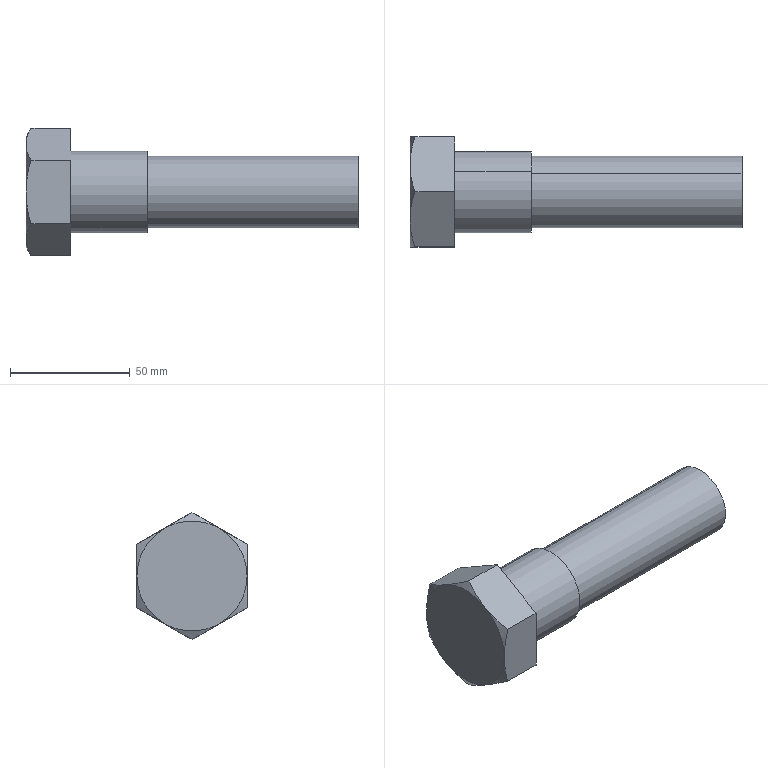Component | SolidWorks | GB_T5782-2016[HexHeadBoltM30_120]-4 | 1 solid | 20 faces | box 138.7 x 46 x 53.12 mm | volume 125419 mm3 | plane 10 | cone 6 | cylinder 4 | commonest cylinder face diameters 30 x2 34 x2
build123d program:
from build123d import *

# Parameters (mm, degrees)
BASE_EXTRUDE_DEPTH  = 18.7
SKETCH8_R           = 17
BOSS_EXTRUDE2_DEPTH = 32


with BuildPart() as part:
    # Sketch1 → Base-Extrude (new body)
    with BuildSketch(Plane(origin=(0, 0, 0), x_dir=(0, 0, -1), z_dir=(1, 0, 0))):
        Polygon((23, 13.279), (23, -13.279), (0, -26.558), (-23, -13.279), (-23, 13.279), (0, 26.558), align=None)
    extrude(amount=BASE_EXTRUDE_DEPTH)

    # Sketch2 → Revolve1 (revolve)
    with BuildSketch(Plane.XY, mode=Mode.PRIVATE) as revolve1_sk:
        Polygon((0, 0), (138.7, 0), (138.7, 11.969), (138.7, 15), (72.7, 15), (0, 15), align=None)
    revolve(revolve1_sk.sketch.rotate(Axis((0, 0, 0), (1, 0, 0)), 90), axis=Axis((0, 0, 0), (1, 0, 0)))

    # Sketch3 → Cut-Revolve1 (revolve, cut)
    with BuildSketch(Plane.XY):
        Polygon((0, 23), (4.941, 31.558), (4.941, 36.558), (-10, 36.558), (-10, 23), align=None)
    revolve(axis=Axis((0, 0, 0), (1, 0, 0)), mode=Mode.SUBTRACT)

    # Sketch8 → Boss-Extrude2 (add)
    with BuildSketch(Plane(origin=(18.7, 0, 0), x_dir=(0, 0, -1), z_dir=(1, 0, 0))):
        Circle(SKETCH8_R)
    extrude(amount=BOSS_EXTRUDE2_DEPTH)


solid = part.part

# Placed as in the assembly
solid = solid.moved(Location((-218.2, -220, 64), (90, 0, 0)))
STEP:
#1=CARTESIAN_POINT('',(-3.13,-8.366,3.031));
#2=VERTEX_POINT('',#1);
#3=CARTESIAN_POINT('',(-3.13,-8.957,2.008));
#4=VERTEX_POINT('',#3);
#5=CARTESIAN_POINT('',(-3.13,-8.661,2.52));
#6=DIRECTION('',(-1.,0.,0.));
#7=DIRECTION('',(0.,0.5,0.866));
#8=AXIS2_PLACEMENT_3D('',#5,#6,#7);
#9=CIRCLE('',#8,0.5906);
#10=EDGE_CURVE('',#2,#4,#9,.T.);
#11=ORIENTED_EDGE('',*,*,#10,.T.);
#12=CARTESIAN_POINT('',(-6.594,-8.957,2.008));
#13=VERTEX_POINT('',#12);
#14=CARTESIAN_POINT('',(-8.591,-8.957,2.008));
#15=DIRECTION('',(-1.,0.,0.));
#16=VECTOR('',#15,39.37);
#17=LINE('',#14,#16);
#18=EDGE_CURVE('',#4,#13,#17,.T.);
#19=ORIENTED_EDGE('',*,*,#18,.T.);
#20=CARTESIAN_POINT('',(-6.594,-8.366,3.031));
#21=VERTEX_POINT('',#20);
#22=CARTESIAN_POINT('',(-6.594,-8.661,2.52));
#23=DIRECTION('',(1.,0.,0.));
#24=DIRECTION('',(0.,-0.5,-0.866));
#25=AXIS2_PLACEMENT_3D('',#22,#23,#24);
#26=CIRCLE('',#25,0.5906);
#27=EDGE_CURVE('',#13,#21,#26,.T.);
#28=ORIENTED_EDGE('',*,*,#27,.T.);
#29=CARTESIAN_POINT('',(-8.591,-8.366,3.031));
#30=DIRECTION('',(-1.,0.,0.));
#31=VECTOR('',#30,39.37);
#32=LINE('',#29,#31);
#33=EDGE_CURVE('',#2,#21,#32,.T.);
#34=ORIENTED_EDGE('',*,*,#33,.F.);
#35=EDGE_LOOP('',(#11,#19,#28,#34));
#36=FACE_OUTER_BOUND('',#35,.T.);
#37=CARTESIAN_POINT('',(-8.591,-8.661,2.52));
#38=DIRECTION('',(-1.,0.,0.));
#39=DIRECTION('',(0.,0.5,0.866));
#40=AXIS2_PLACEMENT_3D('',#37,#38,#39);
#41=CYLINDRICAL_SURFACE('',#40,0.5906);
#42=ADVANCED_FACE('',(#36),#41,.T.);
#43=CARTESIAN_POINT('',(-6.594,-8.996,1.94));
#44=VERTEX_POINT('',#43);
#45=CARTESIAN_POINT('',(-6.594,-8.327,3.099));
#46=VERTEX_POINT('',#45);
#47=CARTESIAN_POINT('',(-6.594,-8.661,2.52));
#48=DIRECTION('',(1.,0.,0.));
#49=DIRECTION('',(0.,-0.5,-0.866));
#50=AXIS2_PLACEMENT_3D('',#47,#48,#49);
#51=CIRCLE('',#50,0.6693);
#52=EDGE_CURVE('',#44,#46,#51,.T.);
#53=ORIENTED_EDGE('',*,*,#52,.F.);
#54=CARTESIAN_POINT('',(-7.854,-8.996,1.94));
#55=VERTEX_POINT('',#54);
#56=CARTESIAN_POINT('',(-6.594,-8.996,1.94));
#57=DIRECTION('',(-1.,0.,0.));
#58=VECTOR('',#57,39.37);
#59=LINE('',#56,#58);
#60=EDGE_CURVE('',#44,#55,#59,.T.);
#61=ORIENTED_EDGE('',*,*,#60,.T.);
#62=CARTESIAN_POINT('',(-7.854,-8.327,3.099));
#63=VERTEX_POINT('',#62);
#64=CARTESIAN_POINT('',(-7.854,-8.661,2.52));
#65=DIRECTION('',(1.,0.,0.));
#66=DIRECTION('',(0.,-0.5,-0.866));
#67=AXIS2_PLACEMENT_3D('',#64,#65,#66);
#68=CIRCLE('',#67,0.6693);
#69=EDGE_CURVE('',#55,#63,#68,.T.);
#70=ORIENTED_EDGE('',*,*,#69,.T.);
#71=CARTESIAN_POINT('',(-6.594,-8.327,3.099));
#72=DIRECTION('',(-1.,0.,0.));
#73=VECTOR('',#72,39.37);
#74=LINE('',#71,#73);
#75=EDGE_CURVE('',#46,#63,#74,.T.);
#76=ORIENTED_EDGE('',*,*,#75,.F.);
#77=EDGE_LOOP('',(#53,#61,#70,#76));
#78=FACE_OUTER_BOUND('',#77,.T.);
#79=CARTESIAN_POINT('',(-6.594,-8.661,2.52));
#80=DIRECTION('',(-1.,0.,0.));
#81=DIRECTION('',(0.,0.5,0.866));
#82=AXIS2_PLACEMENT_3D('',#79,#80,#81);
#83=CYLINDRICAL_SURFACE('',#82,0.6693);
#84=ADVANCED_FACE('',(#78),#83,.T.);
#85=CARTESIAN_POINT('',(-8.51,-7.756,1.997));
#86=VERTEX_POINT('',#85);
#87=CARTESIAN_POINT('',(-8.591,-8.209,1.735));
#88=VERTEX_POINT('',#87);
#89=CARTESIAN_POINT('',(-8.51,-7.756,1.997));
#90=CARTESIAN_POINT('',(-8.534,-7.83,1.954));
#91=CARTESIAN_POINT('',(-8.555,-7.905,1.911));
#92=CARTESIAN_POINT('',(-8.583,-8.055,1.824));
#93=CARTESIAN_POINT('',(-8.591,-8.132,1.78));
#94=CARTESIAN_POINT('',(-8.591,-8.209,1.735));
#95=B_SPLINE_CURVE_WITH_KNOTS('',3,(#89,#90,#91,#92,#93,#94),.UNSPECIFIED.,.F.,.F.,(4,2,4),(0.00000024,0.006718,0.01344),.UNSPECIFIED.);
#96=EDGE_CURVE('',#86,#88,#95,.T.);
#97=ORIENTED_EDGE('',*,*,#96,.F.);
#98=CARTESIAN_POINT('',(-7.854,-7.756,1.997));
#99=VERTEX_POINT('',#98);
#100=CARTESIAN_POINT('',(-7.854,-7.756,1.997));
#101=DIRECTION('',(-1.,0.,0.));
#102=VECTOR('',#101,39.37);
#103=LINE('',#100,#102);
#104=EDGE_CURVE('',#99,#86,#103,.T.);
#105=ORIENTED_EDGE('',*,*,#104,.F.);
#106=CARTESIAN_POINT('',(-7.854,-8.661,1.474));
#107=VERTEX_POINT('',#106);
#108=CARTESIAN_POINT('',(-7.854,-8.661,1.474));
#109=DIRECTION('',(0.,0.866,0.5));
#110=VECTOR('',#109,39.37);
#111=LINE('',#108,#110);
#112=EDGE_CURVE('',#107,#99,#111,.T.);
#113=ORIENTED_EDGE('',*,*,#112,.F.);
#114=CARTESIAN_POINT('',(-8.51,-8.661,1.474));
#115=VERTEX_POINT('',#114);
#116=CARTESIAN_POINT('',(-7.854,-8.661,1.474));
#117=DIRECTION('',(-1.,0.,0.));
#118=VECTOR('',#117,39.37);
#119=LINE('',#116,#118);
#120=EDGE_CURVE('',#107,#115,#119,.T.);
#121=ORIENTED_EDGE('',*,*,#120,.T.);
#122=CARTESIAN_POINT('',(-8.591,-8.209,1.735));
#123=CARTESIAN_POINT('',(-8.591,-8.228,1.724));
#124=CARTESIAN_POINT('',(-8.59,-8.247,1.713));
#125=CARTESIAN_POINT('',(-8.588,-8.286,1.691));
#126=CARTESIAN_POINT('',(-8.587,-8.305,1.68));
#127=CARTESIAN_POINT('',(-8.581,-8.362,1.647));
#128=CARTESIAN_POINT('',(-8.576,-8.4,1.625));
#129=CARTESIAN_POINT('',(-8.555,-8.513,1.56));
#130=CARTESIAN_POINT('',(-8.534,-8.588,1.517));
#131=CARTESIAN_POINT('',(-8.51,-8.661,1.474));
#132=B_SPLINE_CURVE_WITH_KNOTS('',3,(#122,#123,#124,#125,#126,#127,#128,#129,#130,#131),.UNSPECIFIED.,.F.,.F.,(4,2,2,2,4),(0.01344,0.01511,0.01678,0.02013,0.02682),.UNSPECIFIED.);
#133=EDGE_CURVE('',#88,#115,#132,.T.);
#134=ORIENTED_EDGE('',*,*,#133,.F.);
#135=EDGE_LOOP('',(#97,#105,#113,#121,#134));
#136=FACE_OUTER_BOUND('',#135,.T.);
#137=CARTESIAN_POINT('',(-7.854,-8.661,1.474));
#138=DIRECTION('',(0.,-0.5,0.866));
#139=DIRECTION('',(0.,-0.866,-0.5));
#140=AXIS2_PLACEMENT_3D('',#137,#138,#139);
#141=PLANE('',#140);
#142=ADVANCED_FACE('',(#136),#141,.F.);
#143=CARTESIAN_POINT('',(-8.51,-7.756,3.042));
#144=VERTEX_POINT('',#143);
#145=CARTESIAN_POINT('',(-8.591,-7.756,2.52));
#146=VERTEX_POINT('',#145);
#147=CARTESIAN_POINT('',(-8.51,-7.756,3.042));
#148=CARTESIAN_POINT('',(-8.534,-7.756,2.957));
#149=CARTESIAN_POINT('',(-8.555,-7.756,2.871));
#150=CARTESIAN_POINT('',(-8.583,-7.756,2.697));
#151=CARTESIAN_POINT('',(-8.591,-7.756,2.609));
#152=CARTESIAN_POINT('',(-8.591,-7.756,2.52));
#153=B_SPLINE_CURVE_WITH_KNOTS('',3,(#147,#148,#149,#150,#151,#152),.UNSPECIFIED.,.F.,.F.,(4,2,4),(0.00000024,0.006718,0.01344),.UNSPECIFIED.);
#154=EDGE_CURVE('',#144,#146,#153,.T.);
#155=ORIENTED_EDGE('',*,*,#154,.F.);
#156=CARTESIAN_POINT('',(-7.854,-7.756,3.042));
#157=VERTEX_POINT('',#156);
#158=CARTESIAN_POINT('',(-7.854,-7.756,3.042));
#159=DIRECTION('',(-1.,0.,0.));
#160=VECTOR('',#159,39.37);
#161=LINE('',#158,#160);
#162=EDGE_CURVE('',#157,#144,#161,.T.);
#163=ORIENTED_EDGE('',*,*,#162,.F.);
#164=CARTESIAN_POINT('',(-7.854,-7.756,1.997));
#165=DIRECTION('',(0.,0.,1.));
#166=VECTOR('',#165,39.37);
#167=LINE('',#164,#166);
#168=EDGE_CURVE('',#99,#157,#167,.T.);
#169=ORIENTED_EDGE('',*,*,#168,.F.);
#170=ORIENTED_EDGE('',*,*,#104,.T.);
#171=CARTESIAN_POINT('',(-8.591,-7.756,2.52));
#172=CARTESIAN_POINT('',(-8.591,-7.756,2.498));
#173=CARTESIAN_POINT('',(-8.59,-7.756,2.475));
#174=CARTESIAN_POINT('',(-8.588,-7.756,2.431));
#175=CARTESIAN_POINT('',(-8.587,-7.756,2.409));
#176=CARTESIAN_POINT('',(-8.581,-7.756,2.343));
#177=CARTESIAN_POINT('',(-8.576,-7.756,2.299));
#178=CARTESIAN_POINT('',(-8.555,-7.756,2.168));
#179=CARTESIAN_POINT('',(-8.534,-7.756,2.082));
#180=CARTESIAN_POINT('',(-8.51,-7.756,1.997));
#181=B_SPLINE_CURVE_WITH_KNOTS('',3,(#171,#172,#173,#174,#175,#176,#177,#178,#179,#180),.UNSPECIFIED.,.F.,.F.,(4,2,2,2,4),(0.01344,0.01511,0.01678,0.02013,0.02682),.UNSPECIFIED.);
#182=EDGE_CURVE('',#146,#86,#181,.T.);
#183=ORIENTED_EDGE('',*,*,#182,.F.);
#184=EDGE_LOOP('',(#155,#163,#169,#170,#183));
#185=FACE_OUTER_BOUND('',#184,.T.);
#186=CARTESIAN_POINT('',(-7.854,-7.756,1.997));
#187=DIRECTION('',(0.,-1.,0.));
#188=DIRECTION('',(0.,-0.,-1.));
#189=AXIS2_PLACEMENT_3D('',#186,#187,#188);
#190=PLANE('',#189);
#191=ADVANCED_FACE('',(#185),#190,.F.);
#192=CARTESIAN_POINT('',(-8.51,-8.661,3.565));
#193=VERTEX_POINT('',#192);
#194=CARTESIAN_POINT('',(-8.591,-8.209,3.304));
#195=VERTEX_POINT('',#194);
#196=CARTESIAN_POINT('',(-8.51,-8.661,3.565));
#197=CARTESIAN_POINT('',(-8.522,-8.625,3.544));
#198=CARTESIAN_POINT('',(-8.533,-8.587,3.523));
#199=CARTESIAN_POINT('',(-8.553,-8.512,3.479));
#200=CARTESIAN_POINT('',(-8.562,-8.475,3.457));
#201=CARTESIAN_POINT('',(-8.583,-8.361,3.392));
#202=CARTESIAN_POINT('',(-8.591,-8.285,3.348));
#203=CARTESIAN_POINT('',(-8.591,-8.209,3.304));
#204=B_SPLINE_CURVE_WITH_KNOTS('',3,(#196,#197,#198,#199,#200,#201,#202,#203),.UNSPECIFIED.,.F.,.F.,(4,2,2,4),(0.02414,0.0275,0.03086,0.03758),.UNSPECIFIED.);
#205=EDGE_CURVE('',#193,#195,#204,.T.);
#206=ORIENTED_EDGE('',*,*,#205,.F.);
#207=CARTESIAN_POINT('',(-7.854,-8.661,3.565));
#208=VERTEX_POINT('',#207);
#209=CARTESIAN_POINT('',(-7.854,-8.661,3.565));
#210=DIRECTION('',(-1.,0.,0.));
#211=VECTOR('',#210,39.37);
#212=LINE('',#209,#211);
#213=EDGE_CURVE('',#208,#193,#212,.T.);
#214=ORIENTED_EDGE('',*,*,#213,.F.);
#215=CARTESIAN_POINT('',(-7.854,-7.756,3.042));
#216=DIRECTION('',(0.,-0.866,0.5));
#217=VECTOR('',#216,39.37);
#218=LINE('',#215,#217);
#219=EDGE_CURVE('',#157,#208,#218,.T.);
#220=ORIENTED_EDGE('',*,*,#219,.F.);
#221=ORIENTED_EDGE('',*,*,#162,.T.);
#222=CARTESIAN_POINT('',(-8.591,-8.209,3.304));
#223=CARTESIAN_POINT('',(-8.591,-8.17,3.282));
#224=CARTESIAN_POINT('',(-8.589,-8.132,3.26));
#225=CARTESIAN_POINT('',(-8.581,-8.055,3.215));
#226=CARTESIAN_POINT('',(-8.576,-8.017,3.193));
#227=CARTESIAN_POINT('',(-8.554,-7.903,3.128));
#228=CARTESIAN_POINT('',(-8.534,-7.829,3.085));
#229=CARTESIAN_POINT('',(-8.51,-7.756,3.042));
#230=B_SPLINE_CURVE_WITH_KNOTS('',3,(#222,#223,#224,#225,#226,#227,#228,#229),.UNSPECIFIED.,.F.,.F.,(4,2,2,4),(0.03758,0.04094,0.0443,0.05102),.UNSPECIFIED.);
#231=EDGE_CURVE('',#195,#144,#230,.T.);
#232=ORIENTED_EDGE('',*,*,#231,.F.);
#233=EDGE_LOOP('',(#206,#214,#220,#221,#232));
#234=FACE_OUTER_BOUND('',#233,.T.);
#235=CARTESIAN_POINT('',(-7.854,-7.756,3.042));
#236=DIRECTION('',(0.,-0.5,-0.866));
#237=DIRECTION('',(-1.,0.,0.));
#238=AXIS2_PLACEMENT_3D('',#235,#236,#237);
#239=PLANE('',#238);
#240=ADVANCED_FACE('',(#234),#239,.F.);
#241=CARTESIAN_POINT('',(-8.51,-9.567,3.042));
#242=VERTEX_POINT('',#241);
#243=CARTESIAN_POINT('',(-8.591,-9.114,3.304));
#244=VERTEX_POINT('',#243);
#245=CARTESIAN_POINT('',(-8.51,-9.567,3.042));
#246=CARTESIAN_POINT('',(-8.534,-9.493,3.085));
#247=CARTESIAN_POINT('',(-8.555,-9.418,3.128));
#248=CARTESIAN_POINT('',(-8.583,-9.267,3.215));
#249=CARTESIAN_POINT('',(-8.591,-9.191,3.259));
#250=CARTESIAN_POINT('',(-8.591,-9.114,3.304));
#251=B_SPLINE_CURVE_WITH_KNOTS('',3,(#245,#246,#247,#248,#249,#250),.UNSPECIFIED.,.F.,.F.,(4,2,4),(0.00000024,0.006718,0.01344),.UNSPECIFIED.);
#252=EDGE_CURVE('',#242,#244,#251,.T.);
#253=ORIENTED_EDGE('',*,*,#252,.F.);
#254=CARTESIAN_POINT('',(-7.854,-9.567,3.042));
#255=VERTEX_POINT('',#254);
#256=CARTESIAN_POINT('',(-7.854,-9.567,3.042));
#257=DIRECTION('',(-1.,0.,0.));
#258=VECTOR('',#257,39.37);
#259=LINE('',#256,#258);
#260=EDGE_CURVE('',#255,#242,#259,.T.);
#261=ORIENTED_EDGE('',*,*,#260,.F.);
#262=CARTESIAN_POINT('',(-7.854,-9.567,3.042));
#263=DIRECTION('',(0.,-0.866,-0.5));
#264=VECTOR('',#263,39.37);
#265=LINE('',#262,#264);
#266=EDGE_CURVE('',#208,#255,#265,.T.);
#267=ORIENTED_EDGE('',*,*,#266,.F.);
#268=ORIENTED_EDGE('',*,*,#213,.T.);
#269=CARTESIAN_POINT('',(-8.591,-9.114,3.304));
#270=CARTESIAN_POINT('',(-8.591,-9.095,3.315));
#271=CARTESIAN_POINT('',(-8.59,-9.076,3.326));
#272=CARTESIAN_POINT('',(-8.588,-9.037,3.348));
#273=CARTESIAN_POINT('',(-8.587,-9.018,3.359));
#274=CARTESIAN_POINT('',(-8.581,-8.961,3.392));
#275=CARTESIAN_POINT('',(-8.576,-8.923,3.414));
#276=CARTESIAN_POINT('',(-8.555,-8.81,3.48));
#277=CARTESIAN_POINT('',(-8.534,-8.735,3.523));
#278=CARTESIAN_POINT('',(-8.51,-8.661,3.565));
#279=B_SPLINE_CURVE_WITH_KNOTS('',3,(#269,#270,#271,#272,#273,#274,#275,#276,#277,#278),.UNSPECIFIED.,.F.,.F.,(4,2,2,2,4),(0.01344,0.01511,0.01678,0.02013,0.02682),.UNSPECIFIED.);
#280=EDGE_CURVE('',#244,#193,#279,.T.);
#281=ORIENTED_EDGE('',*,*,#280,.F.);
#282=EDGE_LOOP('',(#253,#261,#267,#268,#281));
#283=FACE_OUTER_BOUND('',#282,.T.);
#284=CARTESIAN_POINT('',(-7.854,-9.567,3.042));
#285=DIRECTION('',(0.,0.5,-0.866));
#286=DIRECTION('',(0.,0.866,0.5));
#287=AXIS2_PLACEMENT_3D('',#284,#285,#286);
#288=PLANE('',#287);
#289=ADVANCED_FACE('',(#283),#288,.F.);
#290=CARTESIAN_POINT('',(-8.51,-9.567,1.997));
#291=VERTEX_POINT('',#290);
#292=CARTESIAN_POINT('',(-8.591,-9.567,2.52));
#293=VERTEX_POINT('',#292);
#294=CARTESIAN_POINT('',(-8.51,-9.567,1.997));
#295=CARTESIAN_POINT('',(-8.534,-9.567,2.082));
#296=CARTESIAN_POINT('',(-8.555,-9.567,2.169));
#297=CARTESIAN_POINT('',(-8.583,-9.567,2.343));
#298=CARTESIAN_POINT('',(-8.591,-9.567,2.431));
#299=CARTESIAN_POINT('',(-8.591,-9.567,2.52));
#300=B_SPLINE_CURVE_WITH_KNOTS('',3,(#294,#295,#296,#297,#298,#299),.UNSPECIFIED.,.F.,.F.,(4,2,4),(0.00000024,0.006718,0.01344),.UNSPECIFIED.);
#301=EDGE_CURVE('',#291,#293,#300,.T.);
#302=ORIENTED_EDGE('',*,*,#301,.F.);
#303=CARTESIAN_POINT('',(-7.854,-9.567,1.997));
#304=VERTEX_POINT('',#303);
#305=CARTESIAN_POINT('',(-7.854,-9.567,1.997));
#306=DIRECTION('',(-1.,0.,0.));
#307=VECTOR('',#306,39.37);
#308=LINE('',#305,#307);
#309=EDGE_CURVE('',#304,#291,#308,.T.);
#310=ORIENTED_EDGE('',*,*,#309,.F.);
#311=CARTESIAN_POINT('',(-7.854,-9.567,1.997));
#312=DIRECTION('',(0.,-0.,-1.));
#313=VECTOR('',#312,39.37);
#314=LINE('',#311,#313);
#315=EDGE_CURVE('',#255,#304,#314,.T.);
#316=ORIENTED_EDGE('',*,*,#315,.F.);
#317=ORIENTED_EDGE('',*,*,#260,.T.);
#318=CARTESIAN_POINT('',(-8.591,-9.567,2.52));
#319=CARTESIAN_POINT('',(-8.591,-9.567,2.542));
#320=CARTESIAN_POINT('',(-8.59,-9.567,2.564));
#321=CARTESIAN_POINT('',(-8.588,-9.567,2.609));
#322=CARTESIAN_POINT('',(-8.587,-9.567,2.631));
#323=CARTESIAN_POINT('',(-8.581,-9.567,2.697));
#324=CARTESIAN_POINT('',(-8.576,-9.567,2.741));
#325=CARTESIAN_POINT('',(-8.555,-9.567,2.871));
#326=CARTESIAN_POINT('',(-8.534,-9.567,2.957));
#327=CARTESIAN_POINT('',(-8.51,-9.567,3.042));
#328=B_SPLINE_CURVE_WITH_KNOTS('',3,(#318,#319,#320,#321,#322,#323,#324,#325,#326,#327),.UNSPECIFIED.,.F.,.F.,(4,2,2,2,4),(0.01344,0.01511,0.01678,0.02013,0.02682),.UNSPECIFIED.);
#329=EDGE_CURVE('',#293,#242,#328,.T.);
#330=ORIENTED_EDGE('',*,*,#329,.F.);
#331=EDGE_LOOP('',(#302,#310,#316,#317,#330));
#332=FACE_OUTER_BOUND('',#331,.T.);
#333=CARTESIAN_POINT('',(-7.854,-9.567,1.997));
#334=DIRECTION('',(0.,1.,-0.));
#335=DIRECTION('',(0.,0.,1.));
#336=AXIS2_PLACEMENT_3D('',#333,#334,#335);
#337=PLANE('',#336);
#338=ADVANCED_FACE('',(#332),#337,.F.);
#339=CARTESIAN_POINT('',(-8.591,-9.114,1.735));
#340=VERTEX_POINT('',#339);
#341=CARTESIAN_POINT('',(-8.51,-8.661,1.474));
#342=CARTESIAN_POINT('',(-8.534,-8.735,1.516));
#343=CARTESIAN_POINT('',(-8.554,-8.809,1.559));
#344=CARTESIAN_POINT('',(-8.576,-8.922,1.625));
#345=CARTESIAN_POINT('',(-8.581,-8.96,1.647));
#346=CARTESIAN_POINT('',(-8.589,-9.037,1.691));
#347=CARTESIAN_POINT('',(-8.591,-9.076,1.713));
#348=CARTESIAN_POINT('',(-8.591,-9.114,1.735));
#349=B_SPLINE_CURVE_WITH_KNOTS('',3,(#341,#342,#343,#344,#345,#346,#347,#348),.UNSPECIFIED.,.F.,.F.,(4,2,2,4),(0.05953,0.06625,0.06962,0.07298),.UNSPECIFIED.);
#350=EDGE_CURVE('',#115,#340,#349,.T.);
#351=ORIENTED_EDGE('',*,*,#350,.F.);
#352=ORIENTED_EDGE('',*,*,#120,.F.);
#353=CARTESIAN_POINT('',(-7.854,-8.661,1.474));
#354=DIRECTION('',(0.,0.866,-0.5));
#355=VECTOR('',#354,39.37);
#356=LINE('',#353,#355);
#357=EDGE_CURVE('',#304,#107,#356,.T.);
#358=ORIENTED_EDGE('',*,*,#357,.F.);
#359=ORIENTED_EDGE('',*,*,#309,.T.);
#360=CARTESIAN_POINT('',(-8.591,-9.114,1.735));
#361=CARTESIAN_POINT('',(-8.591,-9.191,1.78));
#362=CARTESIAN_POINT('',(-8.583,-9.267,1.824));
#363=CARTESIAN_POINT('',(-8.562,-9.38,1.889));
#364=CARTESIAN_POINT('',(-8.553,-9.418,1.911));
#365=CARTESIAN_POINT('',(-8.533,-9.493,1.954));
#366=CARTESIAN_POINT('',(-8.522,-9.53,1.976));
#367=CARTESIAN_POINT('',(-8.51,-9.567,1.997));
#368=B_SPLINE_CURVE_WITH_KNOTS('',3,(#360,#361,#362,#363,#364,#365,#366,#367),.UNSPECIFIED.,.F.,.F.,(4,2,2,4),(0.07298,0.07971,0.08307,0.08643),.UNSPECIFIED.);
#369=EDGE_CURVE('',#340,#291,#368,.T.);
#370=ORIENTED_EDGE('',*,*,#369,.F.);
#371=EDGE_LOOP('',(#351,#352,#358,#359,#370));
#372=FACE_OUTER_BOUND('',#371,.T.);
#373=CARTESIAN_POINT('',(-7.854,-8.661,1.474));
#374=DIRECTION('',(0.,0.5,0.866));
#375=DIRECTION('',(0.,-0.866,0.5));
#376=AXIS2_PLACEMENT_3D('',#373,#374,#375);
#377=PLANE('',#376);
#378=ADVANCED_FACE('',(#372),#377,.F.);
#379=CARTESIAN_POINT('',(-7.854,-8.661,2.52));
#380=DIRECTION('',(1.,0.,0.));
#381=DIRECTION('',(0.,-0.5,-0.866));
#382=AXIS2_PLACEMENT_3D('',#379,#380,#381);
#383=CIRCLE('',#382,0.6693);
#384=EDGE_CURVE('',#63,#55,#383,.T.);
#385=ORIENTED_EDGE('',*,*,#384,.F.);
#386=ORIENTED_EDGE('',*,*,#69,.F.);
#387=EDGE_LOOP('',(#385,#386));
#388=FACE_BOUND('',#387,.T.);
#389=ORIENTED_EDGE('',*,*,#112,.T.);
#390=ORIENTED_EDGE('',*,*,#168,.T.);
#391=ORIENTED_EDGE('',*,*,#219,.T.);
#392=ORIENTED_EDGE('',*,*,#266,.T.);
#393=ORIENTED_EDGE('',*,*,#315,.T.);
#394=ORIENTED_EDGE('',*,*,#357,.T.);
#395=EDGE_LOOP('',(#389,#390,#391,#392,#393,#394));
#396=FACE_OUTER_BOUND('',#395,.T.);
#397=CARTESIAN_POINT('',(-7.854,-7.756,1.997));
#398=DIRECTION('',(1.,0.,0.));
#399=DIRECTION('',(0.,-0.5,-0.866));
#400=AXIS2_PLACEMENT_3D('',#397,#398,#399);
#401=PLANE('',#400);
#402=ADVANCED_FACE('',(#388,#396),#401,.T.);
#403=ORIENTED_EDGE('',*,*,#301,.T.);
#404=CARTESIAN_POINT('',(-8.591,-8.661,2.52));
#405=DIRECTION('',(1.,0.,0.));
#406=DIRECTION('',(0.,-0.5,-0.866));
#407=AXIS2_PLACEMENT_3D('',#404,#405,#406);
#408=CIRCLE('',#407,0.9055);
#409=EDGE_CURVE('',#293,#340,#408,.T.);
#410=ORIENTED_EDGE('',*,*,#409,.T.);
#411=ORIENTED_EDGE('',*,*,#369,.T.);
#412=EDGE_LOOP('',(#403,#410,#411));
#413=FACE_OUTER_BOUND('',#412,.T.);
#414=CARTESIAN_POINT('',(-8.591,-8.661,2.52));
#415=DIRECTION('',(1.,0.,0.));
#416=DIRECTION('',(0.,-0.5,-0.866));
#417=AXIS2_PLACEMENT_3D('',#414,#415,#416);
#418=CONICAL_SURFACE('',#417,0.9055,1.047);
#419=ADVANCED_FACE('',(#413),#418,.T.);
#420=ORIENTED_EDGE('',*,*,#252,.T.);
#421=CARTESIAN_POINT('',(-8.591,-8.661,2.52));
#422=DIRECTION('',(1.,0.,0.));
#423=DIRECTION('',(0.,-0.5,-0.866));
#424=AXIS2_PLACEMENT_3D('',#421,#422,#423);
#425=CIRCLE('',#424,0.9055);
#426=EDGE_CURVE('',#244,#293,#425,.T.);
#427=ORIENTED_EDGE('',*,*,#426,.T.);
#428=ORIENTED_EDGE('',*,*,#329,.T.);
#429=EDGE_LOOP('',(#420,#427,#428));
#430=FACE_OUTER_BOUND('',#429,.T.);
#431=CARTESIAN_POINT('',(-8.591,-8.661,2.52));
#432=DIRECTION('',(1.,0.,0.));
#433=DIRECTION('',(0.,-0.5,-0.866));
#434=AXIS2_PLACEMENT_3D('',#431,#432,#433);
#435=CONICAL_SURFACE('',#434,0.9055,1.047);
#436=ADVANCED_FACE('',(#430),#435,.T.);
#437=ORIENTED_EDGE('',*,*,#205,.T.);
#438=CARTESIAN_POINT('',(-8.591,-8.661,2.52));
#439=DIRECTION('',(1.,0.,0.));
#440=DIRECTION('',(0.,-0.5,-0.866));
#441=AXIS2_PLACEMENT_3D('',#438,#439,#440);
#442=CIRCLE('',#441,0.9055);
#443=EDGE_CURVE('',#195,#244,#442,.T.);
#444=ORIENTED_EDGE('',*,*,#443,.T.);
#445=ORIENTED_EDGE('',*,*,#280,.T.);
#446=EDGE_LOOP('',(#437,#444,#445));
#447=FACE_OUTER_BOUND('',#446,.T.);
#448=CARTESIAN_POINT('',(-8.591,-8.661,2.52));
#449=DIRECTION('',(1.,0.,0.));
#450=DIRECTION('',(0.,-0.5,-0.866));
#451=AXIS2_PLACEMENT_3D('',#448,#449,#450);
#452=CONICAL_SURFACE('',#451,0.9055,1.047);
#453=ADVANCED_FACE('',(#447),#452,.T.);
#454=ORIENTED_EDGE('',*,*,#231,.T.);
#455=ORIENTED_EDGE('',*,*,#154,.T.);
#456=CARTESIAN_POINT('',(-8.591,-8.661,2.52));
#457=DIRECTION('',(-1.,0.,0.));
#458=DIRECTION('',(0.,0.5,0.866));
#459=AXIS2_PLACEMENT_3D('',#456,#457,#458);
#460=CIRCLE('',#459,0.9055);
#461=EDGE_CURVE('',#195,#146,#460,.T.);
#462=ORIENTED_EDGE('',*,*,#461,.F.);
#463=EDGE_LOOP('',(#454,#455,#462));
#464=FACE_OUTER_BOUND('',#463,.T.);
#465=CARTESIAN_POINT('',(-8.591,-8.661,2.52));
#466=DIRECTION('',(1.,0.,0.));
#467=DIRECTION('',(0.,-0.5,-0.866));
#468=AXIS2_PLACEMENT_3D('',#465,#466,#467);
#469=CONICAL_SURFACE('',#468,0.9055,1.047);
#470=ADVANCED_FACE('',(#464),#469,.T.);
#471=ORIENTED_EDGE('',*,*,#182,.T.);
#472=ORIENTED_EDGE('',*,*,#96,.T.);
#473=CARTESIAN_POINT('',(-8.591,-8.661,2.52));
#474=DIRECTION('',(1.,0.,0.));
#475=DIRECTION('',(0.,-0.5,-0.866));
#476=AXIS2_PLACEMENT_3D('',#473,#474,#475);
#477=CIRCLE('',#476,0.9055);
#478=EDGE_CURVE('',#88,#146,#477,.T.);
#479=ORIENTED_EDGE('',*,*,#478,.T.);
#480=EDGE_LOOP('',(#471,#472,#479));
#481=FACE_OUTER_BOUND('',#480,.T.);
#482=CARTESIAN_POINT('',(-8.591,-8.661,2.52));
#483=DIRECTION('',(1.,0.,0.));
#484=DIRECTION('',(0.,-0.5,-0.866));
#485=AXIS2_PLACEMENT_3D('',#482,#483,#484);
#486=CONICAL_SURFACE('',#485,0.9055,1.047);
#487=ADVANCED_FACE('',(#481),#486,.T.);
#488=ORIENTED_EDGE('',*,*,#133,.T.);
#489=ORIENTED_EDGE('',*,*,#350,.T.);
#490=CARTESIAN_POINT('',(-8.591,-8.661,2.52));
#491=DIRECTION('',(1.,0.,0.));
#492=DIRECTION('',(0.,-0.5,-0.866));
#493=AXIS2_PLACEMENT_3D('',#490,#491,#492);
#494=CIRCLE('',#493,0.9055);
#495=EDGE_CURVE('',#340,#88,#494,.T.);
#496=ORIENTED_EDGE('',*,*,#495,.T.);
#497=EDGE_LOOP('',(#488,#489,#496));
#498=FACE_OUTER_BOUND('',#497,.T.);
#499=CARTESIAN_POINT('',(-8.591,-8.661,2.52));
#500=DIRECTION('',(1.,0.,0.));
#501=DIRECTION('',(0.,-0.5,-0.866));
#502=AXIS2_PLACEMENT_3D('',#499,#500,#501);
#503=CONICAL_SURFACE('',#502,0.9055,1.047);
#504=ADVANCED_FACE('',(#498),#503,.T.);
#505=ORIENTED_EDGE('',*,*,#495,.F.);
#506=ORIENTED_EDGE('',*,*,#409,.F.);
#507=ORIENTED_EDGE('',*,*,#426,.F.);
#508=ORIENTED_EDGE('',*,*,#443,.F.);
#509=ORIENTED_EDGE('',*,*,#461,.T.);
#510=ORIENTED_EDGE('',*,*,#478,.F.);
#511=EDGE_LOOP('',(#505,#506,#507,#508,#509,#510));
#512=FACE_OUTER_BOUND('',#511,.T.);
#513=CARTESIAN_POINT('',(-8.591,-7.756,1.997));
#514=DIRECTION('',(1.,0.,0.));
#515=DIRECTION('',(0.,-0.5,-0.866));
#516=AXIS2_PLACEMENT_3D('',#513,#514,#515);
#517=PLANE('',#516);
#518=ADVANCED_FACE('',(#512),#517,.F.);
#519=ORIENTED_EDGE('',*,*,#60,.F.);
#520=CARTESIAN_POINT('',(-6.594,-8.661,2.52));
#521=DIRECTION('',(1.,0.,0.));
#522=DIRECTION('',(0.,-0.5,-0.866));
#523=AXIS2_PLACEMENT_3D('',#520,#521,#522);
#524=CIRCLE('',#523,0.6693);
#525=EDGE_CURVE('',#46,#44,#524,.T.);
#526=ORIENTED_EDGE('',*,*,#525,.F.);
#527=ORIENTED_EDGE('',*,*,#75,.T.);
#528=ORIENTED_EDGE('',*,*,#384,.T.);
#529=EDGE_LOOP('',(#519,#526,#527,#528));
#530=FACE_OUTER_BOUND('',#529,.T.);
#531=CARTESIAN_POINT('',(-6.594,-8.661,2.52));
#532=DIRECTION('',(-1.,0.,0.));
#533=DIRECTION('',(0.,0.5,0.866));
#534=AXIS2_PLACEMENT_3D('',#531,#532,#533);
#535=CYLINDRICAL_SURFACE('',#534,0.6693);
#536=ADVANCED_FACE('',(#530),#535,.T.);
#537=CARTESIAN_POINT('',(-6.594,-8.661,2.52));
#538=DIRECTION('',(1.,0.,0.));
#539=DIRECTION('',(0.,-0.5,-0.866));
#540=AXIS2_PLACEMENT_3D('',#537,#538,#539);
#541=CIRCLE('',#540,0.5906);
#542=EDGE_CURVE('',#21,#13,#541,.T.);
#543=ORIENTED_EDGE('',*,*,#542,.F.);
#544=ORIENTED_EDGE('',*,*,#27,.F.);
#545=EDGE_LOOP('',(#543,#544));
#546=FACE_BOUND('',#545,.T.);
#547=ORIENTED_EDGE('',*,*,#525,.T.);
#548=ORIENTED_EDGE('',*,*,#52,.T.);
#549=EDGE_LOOP('',(#547,#548));
#550=FACE_OUTER_BOUND('',#549,.T.);
#551=CARTESIAN_POINT('',(-6.594,-8.661,2.52));
#552=DIRECTION('',(1.,0.,0.));
#553=DIRECTION('',(0.,-0.5,-0.866));
#554=AXIS2_PLACEMENT_3D('',#551,#552,#553);
#555=PLANE('',#554);
#556=ADVANCED_FACE('',(#546,#550),#555,.T.);
#557=ORIENTED_EDGE('',*,*,#10,.F.);
#558=CARTESIAN_POINT('',(-3.13,-8.661,2.52));
#559=DIRECTION('',(-1.,0.,0.));
#560=DIRECTION('',(0.,0.5,0.866));
#561=AXIS2_PLACEMENT_3D('',#558,#559,#560);
#562=CIRCLE('',#561,0.5906);
#563=EDGE_CURVE('',#4,#2,#562,.T.);
#564=ORIENTED_EDGE('',*,*,#563,.F.);
#565=EDGE_LOOP('',(#557,#564));
#566=FACE_OUTER_BOUND('',#565,.T.);
#567=CARTESIAN_POINT('',(-3.13,-8.661,2.52));
#568=DIRECTION('',(-1.,0.,0.));
#569=DIRECTION('',(0.,0.5,0.866));
#570=AXIS2_PLACEMENT_3D('',#567,#568,#569);
#571=PLANE('',#570);
#572=ADVANCED_FACE('',(#566),#571,.F.);
#573=ORIENTED_EDGE('',*,*,#18,.F.);
#574=ORIENTED_EDGE('',*,*,#563,.T.);
#575=ORIENTED_EDGE('',*,*,#33,.T.);
#576=ORIENTED_EDGE('',*,*,#542,.T.);
#577=EDGE_LOOP('',(#573,#574,#575,#576));
#578=FACE_OUTER_BOUND('',#577,.T.);
#579=CARTESIAN_POINT('',(-8.591,-8.661,2.52));
#580=DIRECTION('',(-1.,0.,0.));
#581=DIRECTION('',(0.,0.5,0.866));
#582=AXIS2_PLACEMENT_3D('',#579,#580,#581);
#583=CYLINDRICAL_SURFACE('',#582,0.5906);
#584=ADVANCED_FACE('',(#578),#583,.T.);
#585=CLOSED_SHELL('',(#42,#84,#142,#191,#240,#289,#338,#378,#402,#419,#436,#453,#470,#487,#504,#518,#536,#556,#572,#584));
#586=MANIFOLD_SOLID_BREP('',#585);
#587=CARTESIAN_POINT('',(0.,0.,0.));
#588=DIRECTION('',(0.,0.,1.));
#589=DIRECTION('',(1.,0.,0.));
#590=AXIS2_PLACEMENT_3D('',#587,#588,#589);
#591=(LENGTH_UNIT()NAMED_UNIT(*)SI_UNIT($,.METRE.));
#592=LENGTH_MEASURE_WITH_UNIT(LENGTH_MEASURE(0.0254),#591);
#593=DIMENSIONAL_EXPONENTS(1.,0.,0.,0.,0.,0.,0.);
#594=(CONVERSION_BASED_UNIT('',#592)LENGTH_UNIT()NAMED_UNIT(#593));
#595=UNCERTAINTY_MEASURE_WITH_UNIT(LENGTH_MEASURE(0.00001),#594,'','');
#596=(NAMED_UNIT(*)PLANE_ANGLE_UNIT()SI_UNIT($,.RADIAN.));
#597=(NAMED_UNIT(*)SI_UNIT($,.STERADIAN.)SOLID_ANGLE_UNIT());
#598=(GEOMETRIC_REPRESENTATION_CONTEXT(3)GLOBAL_UNCERTAINTY_ASSIGNED_CONTEXT((#595))GLOBAL_UNIT_ASSIGNED_CONTEXT((#594,#596,#597))REPRESENTATION_CONTEXT('',''));
#599=ADVANCED_BREP_SHAPE_REPRESENTATION('',(#586,#590),#598);
#600=COLOUR_RGB('',0.7922,0.8196,0.9333);
#601=FILL_AREA_STYLE_COLOUR('',#600);
#602=FILL_AREA_STYLE('',(#601));
#603=SURFACE_STYLE_FILL_AREA(#602);
#604=SURFACE_SIDE_STYLE('',(#603));
#605=SURFACE_STYLE_USAGE(.BOTH.,#604);
#606=PRESENTATION_STYLE_ASSIGNMENT((#605));
#607=STYLED_ITEM('',(#606),#586);
#608=PRESENTATION_LAYER_ASSIGNMENT('','',(#607));
#609=(LENGTH_UNIT()NAMED_UNIT(*)SI_UNIT($,.METRE.));
#610=LENGTH_MEASURE_WITH_UNIT(LENGTH_MEASURE(0.0254),#609);
#611=DIMENSIONAL_EXPONENTS(1.,0.,0.,0.,0.,0.,0.);
#612=(CONVERSION_BASED_UNIT('',#610)LENGTH_UNIT()NAMED_UNIT(#611));
#613=UNCERTAINTY_MEASURE_WITH_UNIT(LENGTH_MEASURE(0.00001),#612,'','');
#614=(NAMED_UNIT(*)PLANE_ANGLE_UNIT()SI_UNIT($,.RADIAN.));
#615=(NAMED_UNIT(*)SI_UNIT($,.STERADIAN.)SOLID_ANGLE_UNIT());
#616=(GEOMETRIC_REPRESENTATION_CONTEXT(3)GLOBAL_UNCERTAINTY_ASSIGNED_CONTEXT((#613))GLOBAL_UNIT_ASSIGNED_CONTEXT((#612,#614,#615))REPRESENTATION_CONTEXT('',''));
#617=MECHANICAL_DESIGN_GEOMETRIC_PRESENTATION_REPRESENTATION('',(#607),#616);